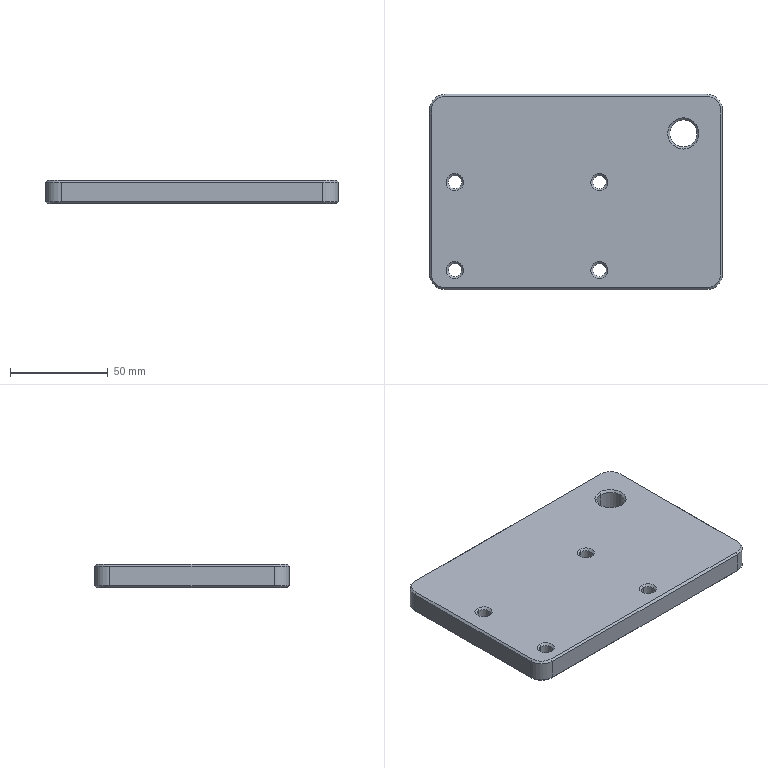Component | SolidWorks | AX00-100.1.1-1_AXFrame_A.1.1-1_AXwheel-assembly-1.1.1-2_AXWHELL-PLATE.1.1-1 | 1 solid | 56 faces | box 150 x 100 x 12 mm | volume 175126 mm3 | cone 28 | cylinder 14 | plane 14 | commonest cylinder face diameters 6.8 x8 16 x4 14 x2
build123d program:
from build123d import *

# Parameters (mm, degrees)
SKETCH1_W            = 100
SKETCH1_H            = 150
BOSS_EXTRUDE1_DEPTH  = 6
M8_TAPPED_HOLE1_D    = 6.8
LPATTERN1_COUNT      = 2
LPATTERN1_PITCH      = 74
LPATTERN1_COUNT_DIR2 = 2
LPATTERN1_PITCH_DIR2 = 45
M16_TAPPED_HOLE1_D   = 14
FILLET1_R            = 8
CHAMFER2_SIZE        = 1


with BuildPart() as part:
    # Sketch1 → Boss-Extrude1 (new, symmetric)
    with BuildSketch(Plane.XY):
        Rectangle(SKETCH1_W, SKETCH1_H)
    extrude(amount=BOSS_EXTRUDE1_DEPTH, both=True)

    # M8 Tapped Hole1 (through all)
    with Locations(Plane(origin=(0, 0, -6), x_dir=(-1, 0, 0), z_dir=(0, 0, -1))):
        with Locations((-5, -62)):
            m8_tapped_hole1 = Hole(M8_TAPPED_HOLE1_D / 2)

    # LPattern1: M8 Tapped Hole1 2 × 2
    with Locations(*[(-j * LPATTERN1_PITCH_DIR2, i * LPATTERN1_PITCH, 0) for i in range(LPATTERN1_COUNT) for j in range(LPATTERN1_COUNT_DIR2) if (i, j) != (0, 0)]):
        add(m8_tapped_hole1, mode=Mode.SUBTRACT)

    # M16 Tapped Hole1 (through all)
    with Locations(Plane(origin=(0, 0, -6), x_dir=(-1, 0, 0), z_dir=(0, 0, -1))):
        with Locations((-30, 55)):
            Hole(M16_TAPPED_HOLE1_D / 2)

    # Fillet1
    fillet1_edges = [part.edges().sort_by_distance(p)[0] for p in [
        (-50, 75, 0),
        (50, 75, 0),
        (50, -75, 0),
        (-50, -75, 0),
    ]]
    fillet(fillet1_edges, radius=FILLET1_R)

    # Chamfer2
    chamfer2_edges = [part.edges().sort_by_distance(p)[0] for p in [
        (1.6, -62, -6),
        (1.6, -62, 6),
        (1.6, 12, -6),
        (1.6, 12, 6),
        (-43.4, -62, 6),
        (-43.4, -62, -6),
        (-43.4, 12, 6),
        (-43.4, 12, -6),
        (23, 55, -6),
        (23, 55, 6),
        (0, -75, -6),
        (0, -75, 6),
        (-50, 0, -6),
        (0, 75, -6),
        (50, 0, -6),
        (47.657, -72.657, -6),
        (47.657, 72.657, -6),
        (-47.657, 72.657, -6),
        (-47.657, -72.657, -6),
        (-50, 0, 6),
        (50, 0, 6),
        (0, 75, 6),
        (47.657, -72.657, 6),
        (47.657, 72.657, 6),
        (-47.657, 72.657, 6),
        (-47.657, -72.657, 6),
    ]]
    chamfer(chamfer2_edges, length=CHAMFER2_SIZE)


solid = part.part

# Placed as in the assembly
solid = solid.moved(Location((-636.369, -336.636, -228.5), (180, 0, -90)))